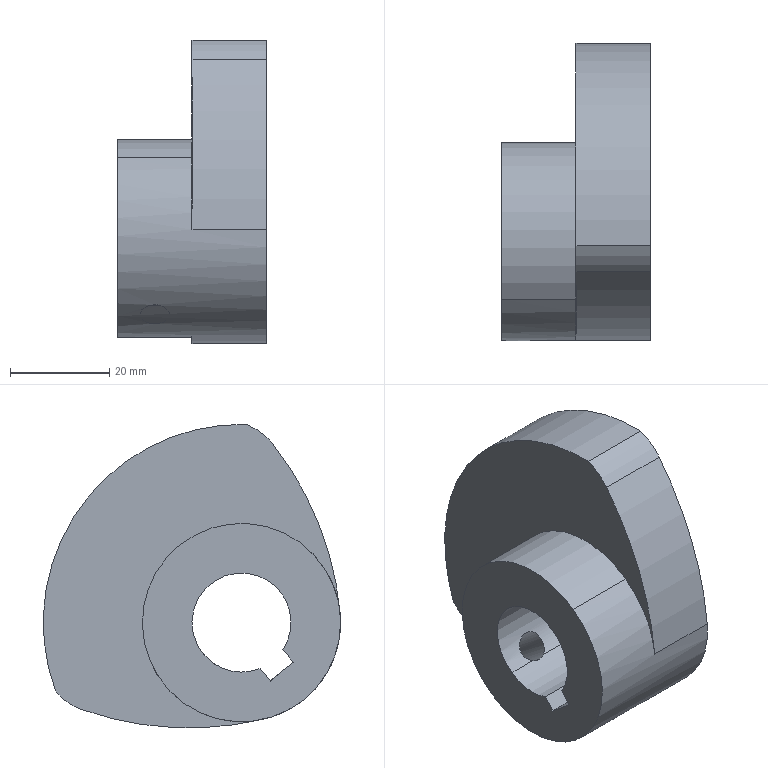Component | SolidWorks | ZL-11-10Cam1-1 | 1 solid | 24 faces | box 30 x 60 x 61.26 mm | volume 51950 mm3 | cylinder 15 | plane 9 | commonest cylinder face diameters 6 x4 20 x3 24 x3 40 x2 130 x2 80 x1
STEP:
#1=CARTESIAN_POINT('',(-5.627,4.744,-0.1471));
#2=VERTEX_POINT('',#1);
#3=CARTESIAN_POINT('',(-5.568,4.608,-0.3201));
#4=VERTEX_POINT('',#3);
#5=CARTESIAN_POINT('',(-5.627,4.744,-0.1471));
#6=CARTESIAN_POINT('',(-5.614,4.744,-0.1471));
#7=CARTESIAN_POINT('',(-5.601,4.743,-0.1493));
#8=CARTESIAN_POINT('',(-5.577,4.74,-0.1572));
#9=CARTESIAN_POINT('',(-5.566,4.737,-0.1631));
#10=CARTESIAN_POINT('',(-5.545,4.73,-0.1775));
#11=CARTESIAN_POINT('',(-5.536,4.726,-0.1862));
#12=CARTESIAN_POINT('',(-5.526,4.718,-0.2001));
#13=CARTESIAN_POINT('',(-5.523,4.715,-0.205));
#14=CARTESIAN_POINT('',(-5.517,4.709,-0.215));
#15=CARTESIAN_POINT('',(-5.515,4.705,-0.2201));
#16=CARTESIAN_POINT('',(-5.512,4.698,-0.2303));
#17=CARTESIAN_POINT('',(-5.51,4.694,-0.2354));
#18=CARTESIAN_POINT('',(-5.509,4.687,-0.2456));
#19=CARTESIAN_POINT('',(-5.509,4.682,-0.2507));
#20=CARTESIAN_POINT('',(-5.51,4.674,-0.2604));
#21=CARTESIAN_POINT('',(-5.511,4.67,-0.2652));
#22=CARTESIAN_POINT('',(-5.514,4.661,-0.2744));
#23=CARTESIAN_POINT('',(-5.516,4.657,-0.2788));
#24=CARTESIAN_POINT('',(-5.52,4.648,-0.2871));
#25=CARTESIAN_POINT('',(-5.523,4.644,-0.291));
#26=CARTESIAN_POINT('',(-5.53,4.636,-0.2984));
#27=CARTESIAN_POINT('',(-5.534,4.632,-0.3018));
#28=CARTESIAN_POINT('',(-5.542,4.624,-0.308));
#29=CARTESIAN_POINT('',(-5.547,4.62,-0.3108));
#30=CARTESIAN_POINT('',(-5.557,4.614,-0.3159));
#31=CARTESIAN_POINT('',(-5.562,4.611,-0.3182));
#32=CARTESIAN_POINT('',(-5.568,4.608,-0.3201));
#33=B_SPLINE_CURVE_WITH_KNOTS('',3,(#5,#6,#7,#8,#9,#10,#11,#12,#13,#14,#15,#16,#17,#18,#19,#20,#21,#22,#23,#24,#25,#26,#27,#28,#29,#30,#31,#32),.UNSPECIFIED.,.F.,.F.,(4,2,2,2,2,2,2,2,2,2,2,2,2,4),(0.009434,0.01041,0.01139,0.01238,0.01287,0.01336,0.01385,0.01434,0.01483,0.01532,0.01581,0.0163,0.01679,0.01728),.UNSPECIFIED.);
#34=EDGE_CURVE('',#2,#4,#33,.T.);
#35=ORIENTED_EDGE('',*,*,#34,.F.);
#36=CARTESIAN_POINT('',(-5.627,5.055,-0.4029));
#37=VERTEX_POINT('',#36);
#38=CARTESIAN_POINT('',(-5.627,5.056,-0.4036));
#39=DIRECTION('',(-0.,0.7727,-0.6348));
#40=VECTOR('',#39,39.37);
#41=LINE('',#38,#40);
#42=EDGE_CURVE('',#2,#37,#41,.T.);
#43=ORIENTED_EDGE('',*,*,#42,.T.);
#44=CARTESIAN_POINT('',(-5.587,5.052,-0.409));
#45=VERTEX_POINT('',#44);
#46=CARTESIAN_POINT('',(-5.587,5.052,-0.409));
#47=CARTESIAN_POINT('',(-5.6,5.054,-0.405));
#48=CARTESIAN_POINT('',(-5.613,5.055,-0.4029));
#49=CARTESIAN_POINT('',(-5.627,5.055,-0.4029));
#50=B_SPLINE_CURVE_WITH_KNOTS('',3,(#46,#47,#48,#49),.UNSPECIFIED.,.F.,.F.,(4,4),(0.,0.001036),.UNSPECIFIED.);
#51=EDGE_CURVE('',#45,#37,#50,.T.);
#52=ORIENTED_EDGE('',*,*,#51,.F.);
#53=CARTESIAN_POINT('',(-5.587,4.911,-0.5807));
#54=VERTEX_POINT('',#53);
#55=CARTESIAN_POINT('',(-5.627,4.981,-0.4948));
#56=DIRECTION('',(-0.,0.7727,-0.6348));
#57=DIRECTION('',(0.,-0.6348,-0.7727));
#58=AXIS2_PLACEMENT_3D('',#55,#56,#57);
#59=CIRCLE('',#58,0.1181);
#60=EDGE_CURVE('',#45,#54,#59,.T.);
#61=ORIENTED_EDGE('',*,*,#60,.T.);
#62=CARTESIAN_POINT('',(-5.627,4.905,-0.5854));
#63=VERTEX_POINT('',#62);
#64=CARTESIAN_POINT('',(-5.627,4.905,-0.5854));
#65=CARTESIAN_POINT('',(-5.613,4.905,-0.5854));
#66=CARTESIAN_POINT('',(-5.6,4.907,-0.5839));
#67=CARTESIAN_POINT('',(-5.587,4.911,-0.5807));
#68=B_SPLINE_CURVE_WITH_KNOTS('',3,(#64,#65,#66,#67),.UNSPECIFIED.,.F.,.F.,(4,4),(0.001036,0.002074),.UNSPECIFIED.);
#69=EDGE_CURVE('',#63,#54,#68,.T.);
#70=ORIENTED_EDGE('',*,*,#69,.F.);
#71=CARTESIAN_POINT('',(-5.627,4.594,-0.3297));
#72=VERTEX_POINT('',#71);
#73=CARTESIAN_POINT('',(-5.627,4.906,-0.5861));
#74=DIRECTION('',(-0.,0.7727,-0.6348));
#75=VECTOR('',#74,39.37);
#76=LINE('',#73,#75);
#77=EDGE_CURVE('',#72,#63,#76,.T.);
#78=ORIENTED_EDGE('',*,*,#77,.F.);
#79=CARTESIAN_POINT('',(-5.568,4.608,-0.3201));
#80=CARTESIAN_POINT('',(-5.572,4.606,-0.3217));
#81=CARTESIAN_POINT('',(-5.577,4.604,-0.3231));
#82=CARTESIAN_POINT('',(-5.586,4.6,-0.3255));
#83=CARTESIAN_POINT('',(-5.591,4.599,-0.3265));
#84=CARTESIAN_POINT('',(-5.606,4.595,-0.3289));
#85=CARTESIAN_POINT('',(-5.617,4.594,-0.3297));
#86=CARTESIAN_POINT('',(-5.627,4.594,-0.3297));
#87=B_SPLINE_CURVE_WITH_KNOTS('',3,(#79,#80,#81,#82,#83,#84,#85,#86),.UNSPECIFIED.,.F.,.F.,(4,2,2,4),(0.01728,0.01767,0.01807,0.01887),.UNSPECIFIED.);
#88=EDGE_CURVE('',#4,#72,#87,.T.);
#89=ORIENTED_EDGE('',*,*,#88,.F.);
#90=EDGE_LOOP('',(#35,#43,#52,#61,#70,#78,#89));
#91=FACE_OUTER_BOUND('',#90,.T.);
#92=CARTESIAN_POINT('',(-5.627,4.981,-0.4948));
#93=DIRECTION('',(-0.,0.7727,-0.6348));
#94=DIRECTION('',(0.,-0.6348,-0.7727));
#95=AXIS2_PLACEMENT_3D('',#92,#93,#94);
#96=CYLINDRICAL_SURFACE('',#95,0.1181);
#97=ADVANCED_FACE('',(#91),#96,.F.);
#98=CARTESIAN_POINT('',(-5.627,4.15,-0.4644));
#99=VERTEX_POINT('',#98);
#100=CARTESIAN_POINT('',(-5.627,3.968,-0.3144));
#101=VERTEX_POINT('',#100);
#102=CARTESIAN_POINT('',(-5.627,4.059,-0.3894));
#103=DIRECTION('',(0.,-0.6348,-0.7727));
#104=DIRECTION('',(0.,-0.7727,0.6348));
#105=AXIS2_PLACEMENT_3D('',#102,#103,#104);
#106=CIRCLE('',#105,0.1181);
#107=EDGE_CURVE('',#99,#101,#106,.T.);
#108=ORIENTED_EDGE('',*,*,#107,.F.);
#109=CARTESIAN_POINT('',(-5.627,3.976,-0.6765));
#110=VERTEX_POINT('',#109);
#111=CARTESIAN_POINT('',(-5.627,3.975,-0.6773));
#112=DIRECTION('',(0.,-0.6348,-0.7727));
#113=VECTOR('',#112,39.37);
#114=LINE('',#111,#113);
#115=EDGE_CURVE('',#99,#110,#114,.T.);
#116=ORIENTED_EDGE('',*,*,#115,.T.);
#117=CARTESIAN_POINT('',(-5.587,3.97,-0.6728));
#118=VERTEX_POINT('',#117);
#119=CARTESIAN_POINT('',(-5.587,3.97,-0.6728));
#120=CARTESIAN_POINT('',(-5.6,3.974,-0.6753));
#121=CARTESIAN_POINT('',(-5.613,3.976,-0.6765));
#122=CARTESIAN_POINT('',(-5.627,3.976,-0.6765));
#123=B_SPLINE_CURVE_WITH_KNOTS('',3,(#119,#120,#121,#122),.UNSPECIFIED.,.F.,.F.,(4,4),(0.,0.001036),.UNSPECIFIED.);
#124=EDGE_CURVE('',#118,#110,#123,.T.);
#125=ORIENTED_EDGE('',*,*,#124,.F.);
#126=CARTESIAN_POINT('',(-5.587,3.798,-0.5318));
#127=VERTEX_POINT('',#126);
#128=CARTESIAN_POINT('',(-5.627,3.884,-0.6023));
#129=DIRECTION('',(0.,-0.6348,-0.7727));
#130=DIRECTION('',(0.,-0.7727,0.6348));
#131=AXIS2_PLACEMENT_3D('',#128,#129,#130);
#132=CIRCLE('',#131,0.1181);
#133=EDGE_CURVE('',#118,#127,#132,.T.);
#134=ORIENTED_EDGE('',*,*,#133,.T.);
#135=CARTESIAN_POINT('',(-5.627,3.793,-0.5265));
#136=VERTEX_POINT('',#135);
#137=CARTESIAN_POINT('',(-5.627,3.793,-0.5265));
#138=CARTESIAN_POINT('',(-5.613,3.793,-0.5265));
#139=CARTESIAN_POINT('',(-5.6,3.795,-0.5283));
#140=CARTESIAN_POINT('',(-5.587,3.798,-0.5318));
#141=B_SPLINE_CURVE_WITH_KNOTS('',3,(#137,#138,#139,#140),.UNSPECIFIED.,.F.,.F.,(4,4),(0.001036,0.002074),.UNSPECIFIED.);
#142=EDGE_CURVE('',#136,#127,#141,.T.);
#143=ORIENTED_EDGE('',*,*,#142,.F.);
#144=CARTESIAN_POINT('',(-5.627,3.793,-0.5273));
#145=DIRECTION('',(0.,-0.6348,-0.7727));
#146=VECTOR('',#145,39.37);
#147=LINE('',#144,#146);
#148=EDGE_CURVE('',#101,#136,#147,.T.);
#149=ORIENTED_EDGE('',*,*,#148,.F.);
#150=EDGE_LOOP('',(#108,#116,#125,#134,#143,#149));
#151=FACE_OUTER_BOUND('',#150,.T.);
#152=CARTESIAN_POINT('',(-5.627,3.884,-0.6023));
#153=DIRECTION('',(0.,-0.6348,-0.7727));
#154=DIRECTION('',(0.,-0.7727,0.6348));
#155=AXIS2_PLACEMENT_3D('',#152,#153,#154);
#156=CYLINDRICAL_SURFACE('',#155,0.1181);
#157=ADVANCED_FACE('',(#151),#156,.F.);
#158=CARTESIAN_POINT('',(-4.741,4.608,-0.3201));
#159=VERTEX_POINT('',#158);
#160=CARTESIAN_POINT('',(-4.741,4.232,-0.3652));
#161=VERTEX_POINT('',#160);
#162=CARTESIAN_POINT('',(-4.741,4.379,0.));
#163=DIRECTION('',(-1.,-0.,0.));
#164=DIRECTION('',(0.,-0.5821,0.8132));
#165=AXIS2_PLACEMENT_3D('',#162,#163,#164);
#166=CIRCLE('',#165,0.3937);
#167=EDGE_CURVE('',#159,#161,#166,.T.);
#168=ORIENTED_EDGE('',*,*,#167,.F.);
#169=CARTESIAN_POINT('',(-4.741,4.608,-0.3201));
#170=DIRECTION('',(-1.,-0.,0.));
#171=VECTOR('',#170,39.37);
#172=LINE('',#169,#171);
#173=EDGE_CURVE('',#159,#4,#172,.T.);
#174=ORIENTED_EDGE('',*,*,#173,.T.);
#175=ORIENTED_EDGE('',*,*,#88,.T.);
#176=CARTESIAN_POINT('',(-5.687,4.608,-0.3201));
#177=VERTEX_POINT('',#176);
#178=CARTESIAN_POINT('',(-5.627,4.594,-0.3297));
#179=CARTESIAN_POINT('',(-5.638,4.594,-0.3297));
#180=CARTESIAN_POINT('',(-5.648,4.595,-0.3289));
#181=CARTESIAN_POINT('',(-5.663,4.599,-0.3265));
#182=CARTESIAN_POINT('',(-5.668,4.6,-0.3255));
#183=CARTESIAN_POINT('',(-5.678,4.604,-0.3231));
#184=CARTESIAN_POINT('',(-5.683,4.606,-0.3217));
#185=CARTESIAN_POINT('',(-5.687,4.608,-0.3201));
#186=B_SPLINE_CURVE_WITH_KNOTS('',3,(#178,#179,#180,#181,#182,#183,#184,#185),.UNSPECIFIED.,.F.,.F.,(4,2,2,4),(0.,0.0007943,0.001192,0.001589),.UNSPECIFIED.);
#187=EDGE_CURVE('',#72,#177,#186,.T.);
#188=ORIENTED_EDGE('',*,*,#187,.T.);
#189=CARTESIAN_POINT('',(-5.923,4.608,-0.3201));
#190=VERTEX_POINT('',#189);
#191=CARTESIAN_POINT('',(-4.741,4.608,-0.3201));
#192=DIRECTION('',(-1.,-0.,0.));
#193=VECTOR('',#192,39.37);
#194=LINE('',#191,#193);
#195=EDGE_CURVE('',#177,#190,#194,.T.);
#196=ORIENTED_EDGE('',*,*,#195,.T.);
#197=CARTESIAN_POINT('',(-5.923,4.232,-0.3652));
#198=VERTEX_POINT('',#197);
#199=CARTESIAN_POINT('',(-5.923,4.379,0.));
#200=DIRECTION('',(-1.,-0.,0.));
#201=DIRECTION('',(0.,-0.5821,0.8132));
#202=AXIS2_PLACEMENT_3D('',#199,#200,#201);
#203=CIRCLE('',#202,0.3937);
#204=EDGE_CURVE('',#190,#198,#203,.T.);
#205=ORIENTED_EDGE('',*,*,#204,.T.);
#206=CARTESIAN_POINT('',(-4.741,4.232,-0.3652));
#207=DIRECTION('',(-1.,-0.,0.));
#208=VECTOR('',#207,39.37);
#209=LINE('',#206,#208);
#210=EDGE_CURVE('',#161,#198,#209,.T.);
#211=ORIENTED_EDGE('',*,*,#210,.F.);
#212=EDGE_LOOP('',(#168,#174,#175,#188,#196,#205,#211));
#213=FACE_OUTER_BOUND('',#212,.T.);
#214=CARTESIAN_POINT('',(-4.741,4.379,0.));
#215=DIRECTION('',(-1.,-0.,0.));
#216=DIRECTION('',(0.,-0.5821,0.8132));
#217=AXIS2_PLACEMENT_3D('',#214,#215,#216);
#218=CYLINDRICAL_SURFACE('',#217,0.3937);
#219=ADVANCED_FACE('',(#213),#218,.F.);
#220=ORIENTED_EDGE('',*,*,#173,.F.);
#221=CARTESIAN_POINT('',(-4.741,4.15,0.3201));
#222=VERTEX_POINT('',#221);
#223=CARTESIAN_POINT('',(-4.741,4.379,0.));
#224=DIRECTION('',(-1.,-0.,0.));
#225=DIRECTION('',(0.,-0.5821,0.8132));
#226=AXIS2_PLACEMENT_3D('',#223,#224,#225);
#227=CIRCLE('',#226,0.3937);
#228=EDGE_CURVE('',#222,#159,#227,.T.);
#229=ORIENTED_EDGE('',*,*,#228,.F.);
#230=CARTESIAN_POINT('',(-5.923,4.15,0.3201));
#231=VERTEX_POINT('',#230);
#232=CARTESIAN_POINT('',(-4.741,4.15,0.3201));
#233=DIRECTION('',(-1.,-0.,0.));
#234=VECTOR('',#233,39.37);
#235=LINE('',#232,#234);
#236=EDGE_CURVE('',#222,#231,#235,.T.);
#237=ORIENTED_EDGE('',*,*,#236,.T.);
#238=CARTESIAN_POINT('',(-5.923,4.379,0.));
#239=DIRECTION('',(-1.,-0.,0.));
#240=DIRECTION('',(0.,-0.5821,0.8132));
#241=AXIS2_PLACEMENT_3D('',#238,#239,#240);
#242=CIRCLE('',#241,0.3937);
#243=EDGE_CURVE('',#231,#190,#242,.T.);
#244=ORIENTED_EDGE('',*,*,#243,.T.);
#245=ORIENTED_EDGE('',*,*,#195,.F.);
#246=CARTESIAN_POINT('',(-5.687,4.608,-0.3201));
#247=CARTESIAN_POINT('',(-5.692,4.611,-0.3182));
#248=CARTESIAN_POINT('',(-5.698,4.614,-0.3159));
#249=CARTESIAN_POINT('',(-5.708,4.62,-0.3108));
#250=CARTESIAN_POINT('',(-5.712,4.624,-0.308));
#251=CARTESIAN_POINT('',(-5.721,4.632,-0.3018));
#252=CARTESIAN_POINT('',(-5.724,4.636,-0.2984));
#253=CARTESIAN_POINT('',(-5.731,4.644,-0.291));
#254=CARTESIAN_POINT('',(-5.734,4.648,-0.2871));
#255=CARTESIAN_POINT('',(-5.741,4.661,-0.2747));
#256=CARTESIAN_POINT('',(-5.744,4.67,-0.2653));
#257=CARTESIAN_POINT('',(-5.746,4.687,-0.2458));
#258=CARTESIAN_POINT('',(-5.745,4.695,-0.2354));
#259=CARTESIAN_POINT('',(-5.738,4.709,-0.215));
#260=CARTESIAN_POINT('',(-5.732,4.715,-0.2048));
#261=CARTESIAN_POINT('',(-5.718,4.726,-0.1861));
#262=CARTESIAN_POINT('',(-5.709,4.73,-0.1775));
#263=CARTESIAN_POINT('',(-5.689,4.737,-0.1631));
#264=CARTESIAN_POINT('',(-5.677,4.74,-0.1572));
#265=CARTESIAN_POINT('',(-5.653,4.743,-0.1493));
#266=CARTESIAN_POINT('',(-5.64,4.744,-0.1471));
#267=CARTESIAN_POINT('',(-5.627,4.744,-0.1471));
#268=B_SPLINE_CURVE_WITH_KNOTS('',3,(#246,#247,#248,#249,#250,#251,#252,#253,#254,#255,#256,#257,#258,#259,#260,#261,#262,#263,#264,#265,#266,#267),.UNSPECIFIED.,.F.,.F.,(4,2,2,2,2,2,2,2,2,2,4),(0.001589,0.002079,0.002569,0.00306,0.00355,0.004531,0.005511,0.006492,0.007473,0.008453,0.009434),.UNSPECIFIED.);
#269=EDGE_CURVE('',#177,#2,#268,.T.);
#270=ORIENTED_EDGE('',*,*,#269,.T.);
#271=ORIENTED_EDGE('',*,*,#34,.T.);
#272=EDGE_LOOP('',(#220,#229,#237,#244,#245,#270,#271));
#273=FACE_OUTER_BOUND('',#272,.T.);
#274=CARTESIAN_POINT('',(-4.741,4.379,0.));
#275=DIRECTION('',(-1.,-0.,0.));
#276=DIRECTION('',(0.,-0.5821,0.8132));
#277=AXIS2_PLACEMENT_3D('',#274,#275,#276);
#278=CYLINDRICAL_SURFACE('',#277,0.3937);
#279=ADVANCED_FACE('',(#273),#278,.F.);
#280=ORIENTED_EDGE('',*,*,#51,.T.);
#281=CARTESIAN_POINT('',(-5.667,5.052,-0.409));
#282=VERTEX_POINT('',#281);
#283=CARTESIAN_POINT('',(-5.627,5.055,-0.4029));
#284=CARTESIAN_POINT('',(-5.641,5.055,-0.4029));
#285=CARTESIAN_POINT('',(-5.654,5.054,-0.405));
#286=CARTESIAN_POINT('',(-5.667,5.052,-0.409));
#287=B_SPLINE_CURVE_WITH_KNOTS('',3,(#283,#284,#285,#286),.UNSPECIFIED.,.F.,.F.,(4,4),(0.001036,0.002074),.UNSPECIFIED.);
#288=EDGE_CURVE('',#37,#282,#287,.T.);
#289=ORIENTED_EDGE('',*,*,#288,.T.);
#290=CARTESIAN_POINT('',(-5.332,5.052,-0.409));
#291=DIRECTION('',(1.,0.,-0.));
#292=VECTOR('',#291,39.37);
#293=LINE('',#290,#292);
#294=EDGE_CURVE('',#282,#45,#293,.T.);
#295=ORIENTED_EDGE('',*,*,#294,.T.);
#296=EDGE_LOOP('',(#280,#289,#295));
#297=FACE_BOUND('',#296,.T.);
#298=CARTESIAN_POINT('',(-5.667,4.911,-0.5807));
#299=VERTEX_POINT('',#298);
#300=CARTESIAN_POINT('',(-5.667,4.911,-0.5807));
#301=CARTESIAN_POINT('',(-5.654,4.907,-0.5839));
#302=CARTESIAN_POINT('',(-5.641,4.905,-0.5854));
#303=CARTESIAN_POINT('',(-5.627,4.905,-0.5854));
#304=B_SPLINE_CURVE_WITH_KNOTS('',3,(#300,#301,#302,#303),.UNSPECIFIED.,.F.,.F.,(4,4),(0.,0.001036),.UNSPECIFIED.);
#305=EDGE_CURVE('',#299,#63,#304,.T.);
#306=ORIENTED_EDGE('',*,*,#305,.T.);
#307=ORIENTED_EDGE('',*,*,#69,.T.);
#308=CARTESIAN_POINT('',(-5.332,4.911,-0.5807));
#309=DIRECTION('',(-1.,-0.,0.));
#310=VECTOR('',#309,39.37);
#311=LINE('',#308,#310);
#312=EDGE_CURVE('',#54,#299,#311,.T.);
#313=ORIENTED_EDGE('',*,*,#312,.T.);
#314=EDGE_LOOP('',(#306,#307,#313));
#315=FACE_BOUND('',#314,.T.);
#316=CARTESIAN_POINT('',(-5.923,3.92,0.6403));
#317=VERTEX_POINT('',#316);
#318=CARTESIAN_POINT('',(-5.923,4.837,-0.6403));
#319=VERTEX_POINT('',#318);
#320=CARTESIAN_POINT('',(-5.923,4.379,0.));
#321=DIRECTION('',(-1.,-0.,0.));
#322=DIRECTION('',(0.,-0.5821,0.8132));
#323=AXIS2_PLACEMENT_3D('',#320,#321,#322);
#324=CIRCLE('',#323,0.7874);
#325=EDGE_CURVE('',#317,#319,#324,.T.);
#326=ORIENTED_EDGE('',*,*,#325,.F.);
#327=CARTESIAN_POINT('',(-5.332,3.92,0.6403));
#328=VERTEX_POINT('',#327);
#329=CARTESIAN_POINT('',(-5.332,3.92,0.6403));
#330=DIRECTION('',(1.,0.,-0.));
#331=VECTOR('',#330,39.37);
#332=LINE('',#329,#331);
#333=EDGE_CURVE('',#317,#328,#332,.T.);
#334=ORIENTED_EDGE('',*,*,#333,.T.);
#335=CARTESIAN_POINT('',(-5.332,4.837,-0.6403));
#336=VERTEX_POINT('',#335);
#337=CARTESIAN_POINT('',(-5.332,4.379,0.));
#338=DIRECTION('',(-1.,-0.,0.));
#339=DIRECTION('',(0.,-0.5821,0.8132));
#340=AXIS2_PLACEMENT_3D('',#337,#338,#339);
#341=CIRCLE('',#340,0.7874);
#342=EDGE_CURVE('',#328,#336,#341,.T.);
#343=ORIENTED_EDGE('',*,*,#342,.T.);
#344=CARTESIAN_POINT('',(-5.332,4.837,-0.6403));
#345=DIRECTION('',(1.,0.,-0.));
#346=VECTOR('',#345,39.37);
#347=LINE('',#344,#346);
#348=EDGE_CURVE('',#319,#336,#347,.T.);
#349=ORIENTED_EDGE('',*,*,#348,.F.);
#350=EDGE_LOOP('',(#326,#334,#343,#349));
#351=FACE_OUTER_BOUND('',#350,.T.);
#352=CARTESIAN_POINT('',(-5.332,4.379,0.));
#353=DIRECTION('',(1.,0.,-0.));
#354=DIRECTION('',(0.,0.5821,-0.8132));
#355=AXIS2_PLACEMENT_3D('',#352,#353,#354);
#356=CYLINDRICAL_SURFACE('',#355,0.7874);
#357=ADVANCED_FACE('',(#297,#315,#351),#356,.T.);
#358=CARTESIAN_POINT('',(-5.332,5.765,-0.6294));
#359=VERTEX_POINT('',#358);
#360=CARTESIAN_POINT('',(-5.332,5.648,-0.6907));
#361=VERTEX_POINT('',#360);
#362=CARTESIAN_POINT('',(-5.332,5.49,-0.2453));
#363=DIRECTION('',(-1.,-0.,0.));
#364=DIRECTION('',(0.,-0.5821,0.8132));
#365=AXIS2_PLACEMENT_3D('',#362,#363,#364);
#366=CIRCLE('',#365,0.4724);
#367=EDGE_CURVE('',#359,#361,#366,.T.);
#368=ORIENTED_EDGE('',*,*,#367,.F.);
#369=CARTESIAN_POINT('',(-4.741,5.765,-0.6294));
#370=VERTEX_POINT('',#369);
#371=CARTESIAN_POINT('',(-5.332,5.765,-0.6294));
#372=DIRECTION('',(1.,0.,-0.));
#373=VECTOR('',#372,39.37);
#374=LINE('',#371,#373);
#375=EDGE_CURVE('',#359,#370,#374,.T.);
#376=ORIENTED_EDGE('',*,*,#375,.T.);
#377=CARTESIAN_POINT('',(-4.741,5.648,-0.6907));
#378=VERTEX_POINT('',#377);
#379=CARTESIAN_POINT('',(-4.741,5.49,-0.2453));
#380=DIRECTION('',(-1.,-0.,0.));
#381=DIRECTION('',(0.,-0.5821,0.8132));
#382=AXIS2_PLACEMENT_3D('',#379,#380,#381);
#383=CIRCLE('',#382,0.4724);
#384=EDGE_CURVE('',#370,#378,#383,.T.);
#385=ORIENTED_EDGE('',*,*,#384,.T.);
#386=CARTESIAN_POINT('',(-5.332,5.648,-0.6907));
#387=DIRECTION('',(1.,0.,-0.));
#388=VECTOR('',#387,39.37);
#389=LINE('',#386,#388);
#390=EDGE_CURVE('',#361,#378,#389,.T.);
#391=ORIENTED_EDGE('',*,*,#390,.F.);
#392=EDGE_LOOP('',(#368,#376,#385,#391));
#393=FACE_OUTER_BOUND('',#392,.T.);
#394=CARTESIAN_POINT('',(-5.332,5.49,-0.2453));
#395=DIRECTION('',(1.,0.,-0.));
#396=DIRECTION('',(0.,0.5821,-0.8132));
#397=AXIS2_PLACEMENT_3D('',#394,#395,#396);
#398=CYLINDRICAL_SURFACE('',#397,0.4724);
#399=ADVANCED_FACE('',(#393),#398,.T.);
#400=CARTESIAN_POINT('',(-5.923,3.968,-0.3144));
#401=VERTEX_POINT('',#400);
#402=CARTESIAN_POINT('',(-4.741,3.968,-0.3144));
#403=DIRECTION('',(-1.,-0.,0.));
#404=VECTOR('',#403,39.37);
#405=LINE('',#402,#404);
#406=EDGE_CURVE('',#101,#401,#405,.T.);
#407=ORIENTED_EDGE('',*,*,#406,.F.);
#408=CARTESIAN_POINT('',(-5.627,4.059,-0.3894));
#409=DIRECTION('',(0.,-0.6348,-0.7727));
#410=DIRECTION('',(0.,-0.7727,0.6348));
#411=AXIS2_PLACEMENT_3D('',#408,#409,#410);
#412=CIRCLE('',#411,0.1181);
#413=EDGE_CURVE('',#101,#99,#412,.T.);
#414=ORIENTED_EDGE('',*,*,#413,.T.);
#415=CARTESIAN_POINT('',(-5.923,4.15,-0.4644));
#416=VERTEX_POINT('',#415);
#417=CARTESIAN_POINT('',(-4.741,4.15,-0.4644));
#418=DIRECTION('',(-1.,-0.,0.));
#419=VECTOR('',#418,39.37);
#420=LINE('',#417,#419);
#421=EDGE_CURVE('',#99,#416,#420,.T.);
#422=ORIENTED_EDGE('',*,*,#421,.T.);
#423=CARTESIAN_POINT('',(-5.923,4.15,-0.4644));
#424=DIRECTION('',(0.,-0.7727,0.6348));
#425=VECTOR('',#424,39.37);
#426=LINE('',#423,#425);
#427=EDGE_CURVE('',#416,#401,#426,.T.);
#428=ORIENTED_EDGE('',*,*,#427,.T.);
#429=EDGE_LOOP('',(#407,#414,#422,#428));
#430=FACE_OUTER_BOUND('',#429,.T.);
#431=CARTESIAN_POINT('',(-4.741,4.15,-0.4644));
#432=DIRECTION('',(0.,-0.6348,-0.7727));
#433=DIRECTION('',(0.,-0.7727,0.6348));
#434=AXIS2_PLACEMENT_3D('',#431,#432,#433);
#435=PLANE('',#434);
#436=ADVANCED_FACE('',(#430),#435,.F.);
#437=ORIENTED_EDGE('',*,*,#375,.F.);
#438=CARTESIAN_POINT('',(-5.332,5.857,-0.5434));
#439=VERTEX_POINT('',#438);
#440=CARTESIAN_POINT('',(-5.332,5.49,-0.2453));
#441=DIRECTION('',(-1.,-0.,0.));
#442=DIRECTION('',(0.,-0.5821,0.8132));
#443=AXIS2_PLACEMENT_3D('',#440,#441,#442);
#444=CIRCLE('',#443,0.4724);
#445=EDGE_CURVE('',#439,#359,#444,.T.);
#446=ORIENTED_EDGE('',*,*,#445,.F.);
#447=CARTESIAN_POINT('',(-4.741,5.857,-0.5434));
#448=VERTEX_POINT('',#447);
#449=CARTESIAN_POINT('',(-5.332,5.857,-0.5434));
#450=DIRECTION('',(1.,0.,-0.));
#451=VECTOR('',#450,39.37);
#452=LINE('',#449,#451);
#453=EDGE_CURVE('',#439,#448,#452,.T.);
#454=ORIENTED_EDGE('',*,*,#453,.T.);
#455=CARTESIAN_POINT('',(-4.741,5.49,-0.2453));
#456=DIRECTION('',(-1.,-0.,0.));
#457=DIRECTION('',(0.,-0.5821,0.8132));
#458=AXIS2_PLACEMENT_3D('',#455,#456,#457);
#459=CIRCLE('',#458,0.4724);
#460=EDGE_CURVE('',#448,#370,#459,.T.);
#461=ORIENTED_EDGE('',*,*,#460,.T.);
#462=EDGE_LOOP('',(#437,#446,#454,#461));
#463=FACE_OUTER_BOUND('',#462,.T.);
#464=CARTESIAN_POINT('',(-5.332,5.49,-0.2453));
#465=DIRECTION('',(1.,0.,-0.));
#466=DIRECTION('',(0.,0.5821,-0.8132));
#467=AXIS2_PLACEMENT_3D('',#464,#465,#466);
#468=CYLINDRICAL_SURFACE('',#467,0.4724);
#469=ADVANCED_FACE('',(#463),#468,.T.);
#470=CARTESIAN_POINT('',(-4.741,4.194,-0.7654));
#471=VERTEX_POINT('',#470);
#472=CARTESIAN_POINT('',(-4.741,4.795,1.722));
#473=DIRECTION('',(-1.,-0.,0.));
#474=DIRECTION('',(-0.,0.5821,-0.8132));
#475=AXIS2_PLACEMENT_3D('',#472,#473,#474);
#476=CIRCLE('',#475,2.559);
#477=EDGE_CURVE('',#378,#471,#476,.T.);
#478=ORIENTED_EDGE('',*,*,#477,.T.);
#479=CARTESIAN_POINT('',(-5.332,4.194,-0.7654));
#480=VERTEX_POINT('',#479);
#481=CARTESIAN_POINT('',(-5.332,4.194,-0.7654));
#482=DIRECTION('',(1.,0.,-0.));
#483=VECTOR('',#482,39.37);
#484=LINE('',#481,#483);
#485=EDGE_CURVE('',#480,#471,#484,.T.);
#486=ORIENTED_EDGE('',*,*,#485,.F.);
#487=CARTESIAN_POINT('',(-5.332,4.795,1.722));
#488=DIRECTION('',(-1.,-0.,0.));
#489=DIRECTION('',(0.,0.5821,-0.8132));
#490=AXIS2_PLACEMENT_3D('',#487,#488,#489);
#491=CIRCLE('',#490,2.559);
#492=EDGE_CURVE('',#361,#480,#491,.T.);
#493=ORIENTED_EDGE('',*,*,#492,.F.);
#494=ORIENTED_EDGE('',*,*,#390,.T.);
#495=EDGE_LOOP('',(#478,#486,#493,#494));
#496=FACE_OUTER_BOUND('',#495,.T.);
#497=CARTESIAN_POINT('',(-5.332,4.795,1.722));
#498=DIRECTION('',(1.,0.,-0.));
#499=DIRECTION('',(0.,0.5821,-0.8132));
#500=AXIS2_PLACEMENT_3D('',#497,#498,#499);
#501=CYLINDRICAL_SURFACE('',#500,2.559);
#502=ADVANCED_FACE('',(#496),#501,.T.);
#503=ORIENTED_EDGE('',*,*,#333,.F.);
#504=CARTESIAN_POINT('',(-5.923,4.379,0.));
#505=DIRECTION('',(-1.,-0.,0.));
#506=DIRECTION('',(0.,-0.5821,0.8132));
#507=AXIS2_PLACEMENT_3D('',#504,#505,#506);
#508=CIRCLE('',#507,0.7874);
#509=EDGE_CURVE('',#319,#317,#508,.T.);
#510=ORIENTED_EDGE('',*,*,#509,.F.);
#511=ORIENTED_EDGE('',*,*,#348,.T.);
#512=CARTESIAN_POINT('',(-5.332,4.379,0.));
#513=DIRECTION('',(-1.,-0.,0.));
#514=DIRECTION('',(0.,-0.5821,0.8132));
#515=AXIS2_PLACEMENT_3D('',#512,#513,#514);
#516=CIRCLE('',#515,0.7874);
#517=EDGE_CURVE('',#336,#480,#516,.T.);
#518=ORIENTED_EDGE('',*,*,#517,.T.);
#519=ORIENTED_EDGE('',*,*,#485,.T.);
#520=CARTESIAN_POINT('',(-4.741,3.595,0.07166));
#521=VERTEX_POINT('',#520);
#522=CARTESIAN_POINT('',(-4.741,4.379,0.));
#523=DIRECTION('',(-1.,-0.,0.));
#524=DIRECTION('',(0.,-0.5821,0.8132));
#525=AXIS2_PLACEMENT_3D('',#522,#523,#524);
#526=CIRCLE('',#525,0.7874);
#527=EDGE_CURVE('',#471,#521,#526,.T.);
#528=ORIENTED_EDGE('',*,*,#527,.T.);
#529=CARTESIAN_POINT('',(-5.332,3.595,0.07166));
#530=VERTEX_POINT('',#529);
#531=CARTESIAN_POINT('',(-5.332,3.595,0.07166));
#532=DIRECTION('',(1.,0.,-0.));
#533=VECTOR('',#532,39.37);
#534=LINE('',#531,#533);
#535=EDGE_CURVE('',#530,#521,#534,.T.);
#536=ORIENTED_EDGE('',*,*,#535,.F.);
#537=CARTESIAN_POINT('',(-5.332,4.379,0.));
#538=DIRECTION('',(-1.,-0.,0.));
#539=DIRECTION('',(0.,-0.5821,0.8132));
#540=AXIS2_PLACEMENT_3D('',#537,#538,#539);
#541=CIRCLE('',#540,0.7874);
#542=EDGE_CURVE('',#530,#328,#541,.T.);
#543=ORIENTED_EDGE('',*,*,#542,.T.);
#544=EDGE_LOOP('',(#503,#510,#511,#518,#519,#528,#536,#543));
#545=FACE_OUTER_BOUND('',#544,.T.);
#546=CARTESIAN_POINT('',(-5.667,3.798,-0.5318));
#547=VERTEX_POINT('',#546);
#548=CARTESIAN_POINT('',(-5.667,3.798,-0.5318));
#549=CARTESIAN_POINT('',(-5.654,3.795,-0.5283));
#550=CARTESIAN_POINT('',(-5.641,3.793,-0.5265));
#551=CARTESIAN_POINT('',(-5.627,3.793,-0.5265));
#552=B_SPLINE_CURVE_WITH_KNOTS('',3,(#548,#549,#550,#551),.UNSPECIFIED.,.F.,.F.,(4,4),(0.,0.001036),.UNSPECIFIED.);
#553=EDGE_CURVE('',#547,#136,#552,.T.);
#554=ORIENTED_EDGE('',*,*,#553,.T.);
#555=ORIENTED_EDGE('',*,*,#142,.T.);
#556=CARTESIAN_POINT('',(-5.332,3.798,-0.5318));
#557=DIRECTION('',(-1.,-0.,0.));
#558=VECTOR('',#557,39.37);
#559=LINE('',#556,#558);
#560=EDGE_CURVE('',#127,#547,#559,.T.);
#561=ORIENTED_EDGE('',*,*,#560,.T.);
#562=EDGE_LOOP('',(#554,#555,#561));
#563=FACE_BOUND('',#562,.T.);
#564=ORIENTED_EDGE('',*,*,#124,.T.);
#565=CARTESIAN_POINT('',(-5.667,3.97,-0.6728));
#566=VERTEX_POINT('',#565);
#567=CARTESIAN_POINT('',(-5.627,3.976,-0.6765));
#568=CARTESIAN_POINT('',(-5.641,3.976,-0.6765));
#569=CARTESIAN_POINT('',(-5.654,3.974,-0.6753));
#570=CARTESIAN_POINT('',(-5.667,3.97,-0.6728));
#571=B_SPLINE_CURVE_WITH_KNOTS('',3,(#567,#568,#569,#570),.UNSPECIFIED.,.F.,.F.,(4,4),(0.001036,0.002074),.UNSPECIFIED.);
#572=EDGE_CURVE('',#110,#566,#571,.T.);
#573=ORIENTED_EDGE('',*,*,#572,.T.);
#574=CARTESIAN_POINT('',(-5.332,3.97,-0.6728));
#575=DIRECTION('',(1.,0.,-0.));
#576=VECTOR('',#575,39.37);
#577=LINE('',#574,#576);
#578=EDGE_CURVE('',#566,#118,#577,.T.);
#579=ORIENTED_EDGE('',*,*,#578,.T.);
#580=EDGE_LOOP('',(#564,#573,#579));
#581=FACE_BOUND('',#580,.T.);
#582=CARTESIAN_POINT('',(-5.332,4.379,0.));
#583=DIRECTION('',(1.,0.,-0.));
#584=DIRECTION('',(0.,0.5821,-0.8132));
#585=AXIS2_PLACEMENT_3D('',#582,#583,#584);
#586=CYLINDRICAL_SURFACE('',#585,0.7874);
#587=ADVANCED_FACE('',(#545,#563,#581),#586,.T.);
#588=CARTESIAN_POINT('',(-4.741,4.134,1.424));
#589=VERTEX_POINT('',#588);
#590=CARTESIAN_POINT('',(-4.741,6.143,-0.1612));
#591=DIRECTION('',(-1.,-0.,0.));
#592=DIRECTION('',(0.,-0.5821,0.8132));
#593=AXIS2_PLACEMENT_3D('',#590,#591,#592);
#594=CIRCLE('',#593,2.559);
#595=EDGE_CURVE('',#521,#589,#594,.T.);
#596=ORIENTED_EDGE('',*,*,#595,.T.);
#597=CARTESIAN_POINT('',(-5.332,4.134,1.424));
#598=VERTEX_POINT('',#597);
#599=CARTESIAN_POINT('',(-5.332,4.134,1.424));
#600=DIRECTION('',(1.,0.,-0.));
#601=VECTOR('',#600,39.37);
#602=LINE('',#599,#601);
#603=EDGE_CURVE('',#598,#589,#602,.T.);
#604=ORIENTED_EDGE('',*,*,#603,.F.);
#605=CARTESIAN_POINT('',(-5.332,6.143,-0.1612));
#606=DIRECTION('',(-1.,-0.,0.));
#607=DIRECTION('',(0.,-0.5821,0.8132));
#608=AXIS2_PLACEMENT_3D('',#605,#606,#607);
#609=CIRCLE('',#608,2.559);
#610=EDGE_CURVE('',#530,#598,#609,.T.);
#611=ORIENTED_EDGE('',*,*,#610,.F.);
#612=ORIENTED_EDGE('',*,*,#535,.T.);
#613=EDGE_LOOP('',(#596,#604,#611,#612));
#614=FACE_OUTER_BOUND('',#613,.T.);
#615=CARTESIAN_POINT('',(-5.332,6.143,-0.1612));
#616=DIRECTION('',(1.,0.,-0.));
#617=DIRECTION('',(0.,0.5821,-0.8132));
#618=AXIS2_PLACEMENT_3D('',#615,#616,#617);
#619=CYLINDRICAL_SURFACE('',#618,2.559);
#620=ADVANCED_FACE('',(#614),#619,.T.);
#621=CARTESIAN_POINT('',(-4.741,4.341,1.574));
#622=VERTEX_POINT('',#621);
#623=CARTESIAN_POINT('',(-4.741,4.505,1.131));
#624=DIRECTION('',(-1.,-0.,0.));
#625=DIRECTION('',(0.,0.5821,-0.8132));
#626=AXIS2_PLACEMENT_3D('',#623,#624,#625);
#627=CIRCLE('',#626,0.4724);
#628=EDGE_CURVE('',#589,#622,#627,.T.);
#629=ORIENTED_EDGE('',*,*,#628,.T.);
#630=CARTESIAN_POINT('',(-5.332,4.341,1.574));
#631=VERTEX_POINT('',#630);
#632=CARTESIAN_POINT('',(-5.332,4.341,1.574));
#633=DIRECTION('',(1.,0.,-0.));
#634=VECTOR('',#633,39.37);
#635=LINE('',#632,#634);
#636=EDGE_CURVE('',#631,#622,#635,.T.);
#637=ORIENTED_EDGE('',*,*,#636,.F.);
#638=CARTESIAN_POINT('',(-5.332,4.505,1.131));
#639=DIRECTION('',(-1.,-0.,0.));
#640=DIRECTION('',(0.,0.5821,-0.8132));
#641=AXIS2_PLACEMENT_3D('',#638,#639,#640);
#642=CIRCLE('',#641,0.4724);
#643=EDGE_CURVE('',#598,#631,#642,.T.);
#644=ORIENTED_EDGE('',*,*,#643,.F.);
#645=ORIENTED_EDGE('',*,*,#603,.T.);
#646=EDGE_LOOP('',(#629,#637,#644,#645));
#647=FACE_OUTER_BOUND('',#646,.T.);
#648=CARTESIAN_POINT('',(-5.332,4.505,1.131));
#649=DIRECTION('',(1.,0.,-0.));
#650=DIRECTION('',(0.,0.5821,-0.8132));
#651=AXIS2_PLACEMENT_3D('',#648,#649,#650);
#652=CYLINDRICAL_SURFACE('',#651,0.4724);
#653=ADVANCED_FACE('',(#647),#652,.T.);
#654=CARTESIAN_POINT('',(-4.741,4.379,0.));
#655=DIRECTION('',(-1.,-0.,0.));
#656=DIRECTION('',(0.,-0.5821,0.8132));
#657=AXIS2_PLACEMENT_3D('',#654,#655,#656);
#658=CIRCLE('',#657,1.575);
#659=EDGE_CURVE('',#622,#448,#658,.T.);
#660=ORIENTED_EDGE('',*,*,#659,.T.);
#661=ORIENTED_EDGE('',*,*,#453,.F.);
#662=CARTESIAN_POINT('',(-5.332,4.379,0.));
#663=DIRECTION('',(-1.,-0.,0.));
#664=DIRECTION('',(0.,-0.5821,0.8132));
#665=AXIS2_PLACEMENT_3D('',#662,#663,#664);
#666=CIRCLE('',#665,1.575);
#667=EDGE_CURVE('',#631,#439,#666,.T.);
#668=ORIENTED_EDGE('',*,*,#667,.F.);
#669=ORIENTED_EDGE('',*,*,#636,.T.);
#670=EDGE_LOOP('',(#660,#661,#668,#669));
#671=FACE_OUTER_BOUND('',#670,.T.);
#672=CARTESIAN_POINT('',(-5.332,4.379,0.));
#673=DIRECTION('',(1.,0.,-0.));
#674=DIRECTION('',(0.,0.5821,-0.8132));
#675=AXIS2_PLACEMENT_3D('',#672,#673,#674);
#676=CYLINDRICAL_SURFACE('',#675,1.575);
#677=ADVANCED_FACE('',(#671),#676,.T.);
#678=ORIENTED_EDGE('',*,*,#542,.F.);
#679=ORIENTED_EDGE('',*,*,#610,.T.);
#680=ORIENTED_EDGE('',*,*,#643,.T.);
#681=ORIENTED_EDGE('',*,*,#667,.T.);
#682=ORIENTED_EDGE('',*,*,#445,.T.);
#683=ORIENTED_EDGE('',*,*,#367,.T.);
#684=ORIENTED_EDGE('',*,*,#492,.T.);
#685=ORIENTED_EDGE('',*,*,#517,.F.);
#686=ORIENTED_EDGE('',*,*,#342,.F.);
#687=EDGE_LOOP('',(#678,#679,#680,#681,#682,#683,#684,#685,#686));
#688=FACE_OUTER_BOUND('',#687,.T.);
#689=CARTESIAN_POINT('',(-5.332,5.143,0.7384));
#690=DIRECTION('',(-1.,-0.,0.));
#691=DIRECTION('',(0.,-0.5821,0.8132));
#692=AXIS2_PLACEMENT_3D('',#689,#690,#691);
#693=PLANE('',#692);
#694=ADVANCED_FACE('',(#688),#693,.T.);
#695=CARTESIAN_POINT('',(-4.741,3.968,-0.3144));
#696=VERTEX_POINT('',#695);
#697=CARTESIAN_POINT('',(-4.741,4.049,-0.2152));
#698=VERTEX_POINT('',#697);
#699=CARTESIAN_POINT('',(-4.741,4.957,0.8905));
#700=DIRECTION('',(-0.,0.6348,0.7727));
#701=VECTOR('',#700,39.37);
#702=LINE('',#699,#701);
#703=EDGE_CURVE('',#696,#698,#702,.T.);
#704=ORIENTED_EDGE('',*,*,#703,.T.);
#705=CARTESIAN_POINT('',(-4.741,4.379,0.));
#706=DIRECTION('',(-1.,-0.,0.));
#707=DIRECTION('',(0.,-0.5821,0.8132));
#708=AXIS2_PLACEMENT_3D('',#705,#706,#707);
#709=CIRCLE('',#708,0.3937);
#710=EDGE_CURVE('',#698,#222,#709,.T.);
#711=ORIENTED_EDGE('',*,*,#710,.T.);
#712=ORIENTED_EDGE('',*,*,#228,.T.);
#713=ORIENTED_EDGE('',*,*,#167,.T.);
#714=CARTESIAN_POINT('',(-4.741,4.15,-0.4644));
#715=VERTEX_POINT('',#714);
#716=CARTESIAN_POINT('',(-4.741,5.14,0.7406));
#717=DIRECTION('',(0.,-0.6348,-0.7727));
#718=VECTOR('',#717,39.37);
#719=LINE('',#716,#718);
#720=EDGE_CURVE('',#161,#715,#719,.T.);
#721=ORIENTED_EDGE('',*,*,#720,.T.);
#722=CARTESIAN_POINT('',(-4.741,4.153,-0.4665));
#723=DIRECTION('',(0.,-0.7727,0.6348));
#724=VECTOR('',#723,39.37);
#725=LINE('',#722,#724);
#726=EDGE_CURVE('',#715,#696,#725,.T.);
#727=ORIENTED_EDGE('',*,*,#726,.T.);
#728=EDGE_LOOP('',(#704,#711,#712,#713,#721,#727));
#729=FACE_BOUND('',#728,.T.);
#730=ORIENTED_EDGE('',*,*,#460,.F.);
#731=ORIENTED_EDGE('',*,*,#659,.F.);
#732=ORIENTED_EDGE('',*,*,#628,.F.);
#733=ORIENTED_EDGE('',*,*,#595,.F.);
#734=ORIENTED_EDGE('',*,*,#527,.F.);
#735=ORIENTED_EDGE('',*,*,#477,.F.);
#736=ORIENTED_EDGE('',*,*,#384,.F.);
#737=EDGE_LOOP('',(#730,#731,#732,#733,#734,#735,#736));
#738=FACE_OUTER_BOUND('',#737,.T.);
#739=CARTESIAN_POINT('',(-4.741,5.143,0.7384));
#740=DIRECTION('',(-1.,-0.,0.));
#741=DIRECTION('',(0.,-0.5821,0.8132));
#742=AXIS2_PLACEMENT_3D('',#739,#740,#741);
#743=PLANE('',#742);
#744=ADVANCED_FACE('',(#729,#738),#743,.F.);
#745=CARTESIAN_POINT('',(-5.923,4.049,-0.2152));
#746=VERTEX_POINT('',#745);
#747=CARTESIAN_POINT('',(-5.923,4.379,0.));
#748=DIRECTION('',(-1.,-0.,0.));
#749=DIRECTION('',(0.,-0.5821,0.8132));
#750=AXIS2_PLACEMENT_3D('',#747,#748,#749);
#751=CIRCLE('',#750,0.3937);
#752=EDGE_CURVE('',#746,#231,#751,.T.);
#753=ORIENTED_EDGE('',*,*,#752,.F.);
#754=CARTESIAN_POINT('',(-5.923,3.968,-0.3144));
#755=DIRECTION('',(-0.,0.6348,0.7727));
#756=VECTOR('',#755,39.37);
#757=LINE('',#754,#756);
#758=EDGE_CURVE('',#401,#746,#757,.T.);
#759=ORIENTED_EDGE('',*,*,#758,.F.);
#760=ORIENTED_EDGE('',*,*,#427,.F.);
#761=CARTESIAN_POINT('',(-5.923,4.232,-0.3652));
#762=DIRECTION('',(0.,-0.6348,-0.7727));
#763=VECTOR('',#762,39.37);
#764=LINE('',#761,#763);
#765=EDGE_CURVE('',#198,#416,#764,.T.);
#766=ORIENTED_EDGE('',*,*,#765,.F.);
#767=ORIENTED_EDGE('',*,*,#204,.F.);
#768=ORIENTED_EDGE('',*,*,#243,.F.);
#769=EDGE_LOOP('',(#753,#759,#760,#766,#767,#768));
#770=FACE_BOUND('',#769,.T.);
#771=ORIENTED_EDGE('',*,*,#509,.T.);
#772=ORIENTED_EDGE('',*,*,#325,.T.);
#773=EDGE_LOOP('',(#771,#772));
#774=FACE_OUTER_BOUND('',#773,.T.);
#775=CARTESIAN_POINT('',(-5.923,4.379,0.));
#776=DIRECTION('',(-1.,-0.,0.));
#777=DIRECTION('',(0.,-0.5821,0.8132));
#778=AXIS2_PLACEMENT_3D('',#775,#776,#777);
#779=PLANE('',#778);
#780=ADVANCED_FACE('',(#770,#774),#779,.T.);
#781=ORIENTED_EDGE('',*,*,#236,.F.);
#782=ORIENTED_EDGE('',*,*,#710,.F.);
#783=CARTESIAN_POINT('',(-4.741,4.049,-0.2152));
#784=DIRECTION('',(-1.,-0.,0.));
#785=VECTOR('',#784,39.37);
#786=LINE('',#783,#785);
#787=EDGE_CURVE('',#698,#746,#786,.T.);
#788=ORIENTED_EDGE('',*,*,#787,.T.);
#789=ORIENTED_EDGE('',*,*,#752,.T.);
#790=EDGE_LOOP('',(#781,#782,#788,#789));
#791=FACE_OUTER_BOUND('',#790,.T.);
#792=CARTESIAN_POINT('',(-4.741,4.379,0.));
#793=DIRECTION('',(-1.,-0.,0.));
#794=DIRECTION('',(0.,-0.5821,0.8132));
#795=AXIS2_PLACEMENT_3D('',#792,#793,#794);
#796=CYLINDRICAL_SURFACE('',#795,0.3937);
#797=ADVANCED_FACE('',(#791),#796,.F.);
#798=ORIENTED_EDGE('',*,*,#758,.T.);
#799=ORIENTED_EDGE('',*,*,#787,.F.);
#800=ORIENTED_EDGE('',*,*,#703,.F.);
#801=CARTESIAN_POINT('',(-4.741,3.968,-0.3144));
#802=DIRECTION('',(-1.,-0.,0.));
#803=VECTOR('',#802,39.37);
#804=LINE('',#801,#803);
#805=EDGE_CURVE('',#696,#101,#804,.T.);
#806=ORIENTED_EDGE('',*,*,#805,.T.);
#807=ORIENTED_EDGE('',*,*,#406,.T.);
#808=EDGE_LOOP('',(#798,#799,#800,#806,#807));
#809=FACE_OUTER_BOUND('',#808,.T.);
#810=CARTESIAN_POINT('',(-4.741,3.968,-0.3144));
#811=DIRECTION('',(0.,-0.7727,0.6348));
#812=DIRECTION('',(-0.,0.6348,0.7727));
#813=AXIS2_PLACEMENT_3D('',#810,#811,#812);
#814=PLANE('',#813);
#815=ADVANCED_FACE('',(#809),#814,.F.);
#816=CARTESIAN_POINT('',(-4.741,4.15,-0.4644));
#817=DIRECTION('',(-1.,-0.,0.));
#818=VECTOR('',#817,39.37);
#819=LINE('',#816,#818);
#820=EDGE_CURVE('',#715,#99,#819,.T.);
#821=ORIENTED_EDGE('',*,*,#820,.T.);
#822=ORIENTED_EDGE('',*,*,#107,.T.);
#823=ORIENTED_EDGE('',*,*,#805,.F.);
#824=ORIENTED_EDGE('',*,*,#726,.F.);
#825=EDGE_LOOP('',(#821,#822,#823,#824));
#826=FACE_OUTER_BOUND('',#825,.T.);
#827=CARTESIAN_POINT('',(-4.741,4.15,-0.4644));
#828=DIRECTION('',(0.,-0.6348,-0.7727));
#829=DIRECTION('',(0.,-0.7727,0.6348));
#830=AXIS2_PLACEMENT_3D('',#827,#828,#829);
#831=PLANE('',#830);
#832=ADVANCED_FACE('',(#826),#831,.F.);
#833=ORIENTED_EDGE('',*,*,#210,.T.);
#834=ORIENTED_EDGE('',*,*,#765,.T.);
#835=ORIENTED_EDGE('',*,*,#421,.F.);
#836=ORIENTED_EDGE('',*,*,#820,.F.);
#837=ORIENTED_EDGE('',*,*,#720,.F.);
#838=EDGE_LOOP('',(#833,#834,#835,#836,#837));
#839=FACE_OUTER_BOUND('',#838,.T.);
#840=CARTESIAN_POINT('',(-4.741,4.232,-0.3652));
#841=DIRECTION('',(-0.,0.7727,-0.6348));
#842=DIRECTION('',(0.,-0.6348,-0.7727));
#843=AXIS2_PLACEMENT_3D('',#840,#841,#842);
#844=PLANE('',#843);
#845=ADVANCED_FACE('',(#839),#844,.F.);
#846=CARTESIAN_POINT('',(-5.627,3.884,-0.6023));
#847=DIRECTION('',(0.,-0.6348,-0.7727));
#848=DIRECTION('',(0.,-0.7727,0.6348));
#849=AXIS2_PLACEMENT_3D('',#846,#847,#848);
#850=CIRCLE('',#849,0.1181);
#851=EDGE_CURVE('',#547,#566,#850,.T.);
#852=ORIENTED_EDGE('',*,*,#851,.F.);
#853=ORIENTED_EDGE('',*,*,#560,.F.);
#854=ORIENTED_EDGE('',*,*,#133,.F.);
#855=ORIENTED_EDGE('',*,*,#578,.F.);
#856=EDGE_LOOP('',(#852,#853,#854,#855));
#857=FACE_OUTER_BOUND('',#856,.T.);
#858=CARTESIAN_POINT('',(-5.745,3.884,-0.6023));
#859=DIRECTION('',(0.,-0.6348,-0.7727));
#860=DIRECTION('',(0.,-0.7727,0.6348));
#861=AXIS2_PLACEMENT_3D('',#858,#859,#860);
#862=PLANE('',#861);
#863=ADVANCED_FACE('',(#857),#862,.F.);
#864=ORIENTED_EDGE('',*,*,#115,.F.);
#865=ORIENTED_EDGE('',*,*,#413,.F.);
#866=ORIENTED_EDGE('',*,*,#148,.T.);
#867=ORIENTED_EDGE('',*,*,#553,.F.);
#868=ORIENTED_EDGE('',*,*,#851,.T.);
#869=ORIENTED_EDGE('',*,*,#572,.F.);
#870=EDGE_LOOP('',(#864,#865,#866,#867,#868,#869));
#871=FACE_OUTER_BOUND('',#870,.T.);
#872=CARTESIAN_POINT('',(-5.627,3.884,-0.6023));
#873=DIRECTION('',(0.,-0.6348,-0.7727));
#874=DIRECTION('',(0.,-0.7727,0.6348));
#875=AXIS2_PLACEMENT_3D('',#872,#873,#874);
#876=CYLINDRICAL_SURFACE('',#875,0.1181);
#877=ADVANCED_FACE('',(#871),#876,.F.);
#878=CARTESIAN_POINT('',(-5.627,4.981,-0.4948));
#879=DIRECTION('',(-0.,0.7727,-0.6348));
#880=DIRECTION('',(0.,-0.6348,-0.7727));
#881=AXIS2_PLACEMENT_3D('',#878,#879,#880);
#882=CIRCLE('',#881,0.1181);
#883=EDGE_CURVE('',#299,#282,#882,.T.);
#884=ORIENTED_EDGE('',*,*,#883,.F.);
#885=ORIENTED_EDGE('',*,*,#312,.F.);
#886=ORIENTED_EDGE('',*,*,#60,.F.);
#887=ORIENTED_EDGE('',*,*,#294,.F.);
#888=EDGE_LOOP('',(#884,#885,#886,#887));
#889=FACE_OUTER_BOUND('',#888,.T.);
#890=CARTESIAN_POINT('',(-5.745,4.981,-0.4948));
#891=DIRECTION('',(-0.,0.7727,-0.6348));
#892=DIRECTION('',(0.,-0.6348,-0.7727));
#893=AXIS2_PLACEMENT_3D('',#890,#891,#892);
#894=PLANE('',#893);
#895=ADVANCED_FACE('',(#889),#894,.F.);
#896=ORIENTED_EDGE('',*,*,#42,.F.);
#897=ORIENTED_EDGE('',*,*,#269,.F.);
#898=ORIENTED_EDGE('',*,*,#187,.F.);
#899=ORIENTED_EDGE('',*,*,#77,.T.);
#900=ORIENTED_EDGE('',*,*,#305,.F.);
#901=ORIENTED_EDGE('',*,*,#883,.T.);
#902=ORIENTED_EDGE('',*,*,#288,.F.);
#903=EDGE_LOOP('',(#896,#897,#898,#899,#900,#901,#902));
#904=FACE_OUTER_BOUND('',#903,.T.);
#905=CARTESIAN_POINT('',(-5.627,4.981,-0.4948));
#906=DIRECTION('',(-0.,0.7727,-0.6348));
#907=DIRECTION('',(0.,-0.6348,-0.7727));
#908=AXIS2_PLACEMENT_3D('',#905,#906,#907);
#909=CYLINDRICAL_SURFACE('',#908,0.1181);
#910=ADVANCED_FACE('',(#904),#909,.F.);
#911=CLOSED_SHELL('',(#97,#157,#219,#279,#357,#399,#436,#469,#502,#587,#620,#653,#677,#694,#744,#780,#797,#815,#832,#845,#863,#877,#895,#910));
#912=MANIFOLD_SOLID_BREP('',#911);
#913=CARTESIAN_POINT('',(0.,0.,0.));
#914=DIRECTION('',(0.,0.,1.));
#915=DIRECTION('',(1.,0.,0.));
#916=AXIS2_PLACEMENT_3D('',#913,#914,#915);
#917=(LENGTH_UNIT()NAMED_UNIT(*)SI_UNIT($,.METRE.));
#918=LENGTH_MEASURE_WITH_UNIT(LENGTH_MEASURE(0.0254),#917);
#919=DIMENSIONAL_EXPONENTS(1.,0.,0.,0.,0.,0.,0.);
#920=(CONVERSION_BASED_UNIT('',#918)LENGTH_UNIT()NAMED_UNIT(#919));
#921=UNCERTAINTY_MEASURE_WITH_UNIT(LENGTH_MEASURE(0.00001),#920,'','');
#922=(NAMED_UNIT(*)PLANE_ANGLE_UNIT()SI_UNIT($,.RADIAN.));
#923=(NAMED_UNIT(*)SI_UNIT($,.STERADIAN.)SOLID_ANGLE_UNIT());
#924=(GEOMETRIC_REPRESENTATION_CONTEXT(3)GLOBAL_UNCERTAINTY_ASSIGNED_CONTEXT((#921))GLOBAL_UNIT_ASSIGNED_CONTEXT((#920,#922,#923))REPRESENTATION_CONTEXT('',''));
#925=ADVANCED_BREP_SHAPE_REPRESENTATION('',(#912,#916),#924);
#926=COLOUR_RGB('',0.7922,0.8196,0.9333);
#927=FILL_AREA_STYLE_COLOUR('',#926);
#928=FILL_AREA_STYLE('',(#927));
#929=SURFACE_STYLE_FILL_AREA(#928);
#930=SURFACE_SIDE_STYLE('',(#929));
#931=SURFACE_STYLE_USAGE(.BOTH.,#930);
#932=PRESENTATION_STYLE_ASSIGNMENT((#931));
#933=STYLED_ITEM('',(#932),#912);
#934=PRESENTATION_LAYER_ASSIGNMENT('','',(#933));
#935=(LENGTH_UNIT()NAMED_UNIT(*)SI_UNIT($,.METRE.));
#936=LENGTH_MEASURE_WITH_UNIT(LENGTH_MEASURE(0.0254),#935);
#937=DIMENSIONAL_EXPONENTS(1.,0.,0.,0.,0.,0.,0.);
#938=(CONVERSION_BASED_UNIT('',#936)LENGTH_UNIT()NAMED_UNIT(#937));
#939=UNCERTAINTY_MEASURE_WITH_UNIT(LENGTH_MEASURE(0.00001),#938,'','');
#940=(NAMED_UNIT(*)PLANE_ANGLE_UNIT()SI_UNIT($,.RADIAN.));
#941=(NAMED_UNIT(*)SI_UNIT($,.STERADIAN.)SOLID_ANGLE_UNIT());
#942=(GEOMETRIC_REPRESENTATION_CONTEXT(3)GLOBAL_UNCERTAINTY_ASSIGNED_CONTEXT((#939))GLOBAL_UNIT_ASSIGNED_CONTEXT((#938,#940,#941))REPRESENTATION_CONTEXT('',''));
#943=MECHANICAL_DESIGN_GEOMETRIC_PRESENTATION_REPRESENTATION('',(#933),#942);